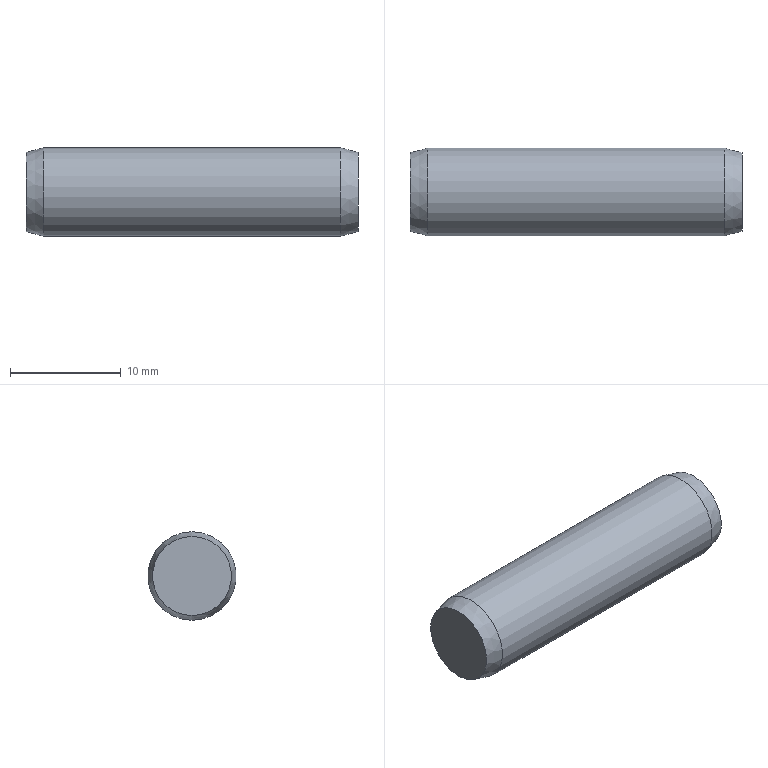Component | NX | GB-T119_1-2000_8X30 | 1 solid | 5 faces | box 30 x 8 x 8 mm | volume 1491 mm3 | plane 2 | cone 2 | cylinder 1 | commonest cylinder face diameters 8 x1
STEP:
#1=CARTESIAN_POINT('',(0.,0.,0.));
#2=DIRECTION('',(0.,0.,1.));
#3=DIRECTION('',(1.,0.,0.));
#4=AXIS2_PLACEMENT_3D('',#1,#2,#3);
#5=CARTESIAN_POINT('',(545.625,96.091,29.014));
#6=VERTEX_POINT('',#5);
#7=CARTESIAN_POINT('',(545.625,96.091,25.443));
#8=DIRECTION('',(-1.,0.,0.));
#9=DIRECTION('',(0.,0.,1.));
#10=AXIS2_PLACEMENT_3D('',#7,#8,#9);
#11=CIRCLE('',#10,3.571);
#12=CARTESIAN_POINT('',(545.625,96.091,25.443));
#13=DIRECTION('',(-1.,0.,0.));
#14=DIRECTION('',(0.,0.,1.));
#15=AXIS2_PLACEMENT_3D('',#12,#13,#14);
#16=PLANE('',#15);
#17=CARTESIAN_POINT('',(0.,0.));
#18=DIRECTION('',(1.,0.));
#19=AXIS2_PLACEMENT_2D('',#17,#18);
#20=CIRCLE('',#19,3.571);
#21=(GEOMETRIC_REPRESENTATION_CONTEXT(2)PARAMETRIC_REPRESENTATION_CONTEXT()REPRESENTATION_CONTEXT('',''));
#22=DEFINITIONAL_REPRESENTATION('',(#20),#21);
#23=PCURVE('',#16,#22);
#24=CARTESIAN_POINT('',(545.625,96.091,25.443));
#25=DIRECTION('',(1.,0.,0.));
#26=DIRECTION('',(0.,0.,-1.));
#27=AXIS2_PLACEMENT_3D('',#24,#25,#26);
#28=CONICAL_SURFACE('',#27,3.571,0.2618);
#29=CARTESIAN_POINT('',(9.425,0.));
#30=DIRECTION('',(-1.,0.));
#31=VECTOR('',#30,1.);
#32=LINE('',#29,#31);
#33=(GEOMETRIC_REPRESENTATION_CONTEXT(2)PARAMETRIC_REPRESENTATION_CONTEXT()REPRESENTATION_CONTEXT('',''));
#34=DEFINITIONAL_REPRESENTATION('',(#32),#33);
#35=PCURVE('',#28,#34);
#36=SURFACE_CURVE('',#11,(#23,#35),.PCURVE_S1.);
#37=EDGE_CURVE('',#6,#6,#36,.T.);
#38=ORIENTED_EDGE('',*,*,#37,.T.);
#39=EDGE_LOOP('',(#38));
#40=FACE_BOUND('',#39,.T.);
#41=ADVANCED_FACE('',(#40),#16,.T.);
#42=CARTESIAN_POINT('',(547.225,96.091,29.443));
#43=VERTEX_POINT('',#42);
#44=CARTESIAN_POINT('',(547.225,96.091,25.443));
#45=DIRECTION('',(-1.,0.,0.));
#46=DIRECTION('',(0.,0.,1.));
#47=AXIS2_PLACEMENT_3D('',#44,#45,#46);
#48=CIRCLE('',#47,4.);
#49=CARTESIAN_POINT('',(9.425,1.6));
#50=DIRECTION('',(-1.,0.));
#51=VECTOR('',#50,1.);
#52=LINE('',#49,#51);
#53=(GEOMETRIC_REPRESENTATION_CONTEXT(2)PARAMETRIC_REPRESENTATION_CONTEXT()REPRESENTATION_CONTEXT('',''));
#54=DEFINITIONAL_REPRESENTATION('',(#52),#53);
#55=PCURVE('',#28,#54);
#56=CARTESIAN_POINT('',(575.625,96.091,25.443));
#57=DIRECTION('',(-1.,0.,0.));
#58=DIRECTION('',(0.,0.,1.));
#59=AXIS2_PLACEMENT_3D('',#56,#57,#58);
#60=CYLINDRICAL_SURFACE('',#59,4.);
#61=CARTESIAN_POINT('',(0.,28.4));
#62=DIRECTION('',(1.,0.));
#63=VECTOR('',#62,1.);
#64=LINE('',#61,#63);
#65=(GEOMETRIC_REPRESENTATION_CONTEXT(2)PARAMETRIC_REPRESENTATION_CONTEXT()REPRESENTATION_CONTEXT('',''));
#66=DEFINITIONAL_REPRESENTATION('',(#64),#65);
#67=PCURVE('',#60,#66);
#68=SURFACE_CURVE('',#48,(#55,#67),.PCURVE_S1.);
#69=EDGE_CURVE('',#43,#43,#68,.T.);
#70=ORIENTED_EDGE('',*,*,#69,.T.);
#71=CARTESIAN_POINT('',(545.625,96.091,29.014));
#72=CARTESIAN_POINT('',(547.225,96.091,29.443));
#73=B_SPLINE_CURVE_WITH_KNOTS('',1,(#71,#72),.UNSPECIFIED.,.F.,.F.,(2,2),(0.,1.656),.PIECEWISE_BEZIER_KNOTS.);
#74=CARTESIAN_POINT('',(3.142,0.));
#75=DIRECTION('',(0.,1.));
#76=VECTOR('',#75,1.);
#77=LINE('',#74,#76);
#78=(GEOMETRIC_REPRESENTATION_CONTEXT(2)PARAMETRIC_REPRESENTATION_CONTEXT()REPRESENTATION_CONTEXT('',''));
#79=DEFINITIONAL_REPRESENTATION('',(#77),#78);
#80=PCURVE('',#28,#79);
#81=CARTESIAN_POINT('',(9.425,0.));
#82=DIRECTION('',(0.,1.));
#83=VECTOR('',#82,1.);
#84=LINE('',#81,#83);
#85=(GEOMETRIC_REPRESENTATION_CONTEXT(2)PARAMETRIC_REPRESENTATION_CONTEXT()REPRESENTATION_CONTEXT('',''));
#86=DEFINITIONAL_REPRESENTATION('',(#84),#85);
#87=PCURVE('',#28,#86);
#88=SEAM_CURVE('',#73,(#80,#87),.PCURVE_S1.);
#89=EDGE_CURVE('',#6,#43,#88,.T.);
#90=ORIENTED_EDGE('',*,*,#89,.F.);
#91=ORIENTED_EDGE('',*,*,#37,.F.);
#92=ORIENTED_EDGE('',*,*,#89,.T.);
#93=EDGE_LOOP('',(#70,#90,#91,#92));
#94=FACE_BOUND('',#93,.T.);
#95=ADVANCED_FACE('',(#94),#28,.T.);
#96=CARTESIAN_POINT('',(574.025,96.091,29.443));
#97=VERTEX_POINT('',#96);
#98=CARTESIAN_POINT('',(574.025,96.091,25.443));
#99=DIRECTION('',(-1.,0.,0.));
#100=DIRECTION('',(0.,0.,1.));
#101=AXIS2_PLACEMENT_3D('',#98,#99,#100);
#102=CIRCLE('',#101,4.);
#103=CARTESIAN_POINT('',(0.,1.6));
#104=DIRECTION('',(1.,0.));
#105=VECTOR('',#104,1.);
#106=LINE('',#103,#105);
#107=(GEOMETRIC_REPRESENTATION_CONTEXT(2)PARAMETRIC_REPRESENTATION_CONTEXT()REPRESENTATION_CONTEXT('',''));
#108=DEFINITIONAL_REPRESENTATION('',(#106),#107);
#109=PCURVE('',#60,#108);
#110=CARTESIAN_POINT('',(574.025,96.091,25.443));
#111=DIRECTION('',(-1.,0.,0.));
#112=DIRECTION('',(0.,0.,1.));
#113=AXIS2_PLACEMENT_3D('',#110,#111,#112);
#114=CONICAL_SURFACE('',#113,4.,0.2618);
#115=CARTESIAN_POINT('',(0.,0.));
#116=DIRECTION('',(1.,0.));
#117=VECTOR('',#116,1.);
#118=LINE('',#115,#117);
#119=(GEOMETRIC_REPRESENTATION_CONTEXT(2)PARAMETRIC_REPRESENTATION_CONTEXT()REPRESENTATION_CONTEXT('',''));
#120=DEFINITIONAL_REPRESENTATION('',(#118),#119);
#121=PCURVE('',#114,#120);
#122=SURFACE_CURVE('',#102,(#109,#121),.PCURVE_S1.);
#123=EDGE_CURVE('',#97,#97,#122,.T.);
#124=ORIENTED_EDGE('',*,*,#123,.T.);
#125=CARTESIAN_POINT('',(574.025,96.091,29.443));
#126=CARTESIAN_POINT('',(547.225,96.091,29.443));
#127=B_SPLINE_CURVE_WITH_KNOTS('',1,(#125,#126),.UNSPECIFIED.,.F.,.F.,(2,2),(1.6,28.4),.PIECEWISE_BEZIER_KNOTS.);
#128=CARTESIAN_POINT('',(6.283,0.));
#129=DIRECTION('',(0.,1.));
#130=VECTOR('',#129,1.);
#131=LINE('',#128,#130);
#132=(GEOMETRIC_REPRESENTATION_CONTEXT(2)PARAMETRIC_REPRESENTATION_CONTEXT()REPRESENTATION_CONTEXT('',''));
#133=DEFINITIONAL_REPRESENTATION('',(#131),#132);
#134=PCURVE('',#60,#133);
#135=CARTESIAN_POINT('',(0.,0.));
#136=DIRECTION('',(0.,1.));
#137=VECTOR('',#136,1.);
#138=LINE('',#135,#137);
#139=(GEOMETRIC_REPRESENTATION_CONTEXT(2)PARAMETRIC_REPRESENTATION_CONTEXT()REPRESENTATION_CONTEXT('',''));
#140=DEFINITIONAL_REPRESENTATION('',(#138),#139);
#141=PCURVE('',#60,#140);
#142=SEAM_CURVE('',#127,(#134,#141),.PCURVE_S1.);
#143=EDGE_CURVE('',#97,#43,#142,.T.);
#144=ORIENTED_EDGE('',*,*,#143,.T.);
#145=ORIENTED_EDGE('',*,*,#69,.F.);
#146=ORIENTED_EDGE('',*,*,#143,.F.);
#147=EDGE_LOOP('',(#124,#144,#145,#146));
#148=FACE_BOUND('',#147,.T.);
#149=ADVANCED_FACE('',(#148),#60,.T.);
#150=CARTESIAN_POINT('',(575.625,96.091,29.014));
#151=VERTEX_POINT('',#150);
#152=CARTESIAN_POINT('',(575.625,96.091,25.443));
#153=DIRECTION('',(-1.,0.,0.));
#154=DIRECTION('',(0.,0.,1.));
#155=AXIS2_PLACEMENT_3D('',#152,#153,#154);
#156=CIRCLE('',#155,3.571);
#157=CARTESIAN_POINT('',(0.,-1.6));
#158=DIRECTION('',(1.,0.));
#159=VECTOR('',#158,1.);
#160=LINE('',#157,#159);
#161=(GEOMETRIC_REPRESENTATION_CONTEXT(2)PARAMETRIC_REPRESENTATION_CONTEXT()REPRESENTATION_CONTEXT('',''));
#162=DEFINITIONAL_REPRESENTATION('',(#160),#161);
#163=PCURVE('',#114,#162);
#164=CARTESIAN_POINT('',(575.625,96.091,21.872));
#165=DIRECTION('',(1.,0.,0.));
#166=DIRECTION('',(0.,0.,-1.));
#167=AXIS2_PLACEMENT_3D('',#164,#165,#166);
#168=PLANE('',#167);
#169=CARTESIAN_POINT('',(-7.143,0.));
#170=CARTESIAN_POINT('',(-7.143,6.186));
#171=CARTESIAN_POINT('',(-1.786,3.093));
#172=CARTESIAN_POINT('',(3.571,0.));
#173=CARTESIAN_POINT('',(-1.786,-3.093));
#174=CARTESIAN_POINT('',(-7.143,-6.186));
#175=CARTESIAN_POINT('',(-7.143,0.));
#176=(BOUNDED_CURVE()B_SPLINE_CURVE(2,(#169,#170,#171,#172,#173,#174,#175),.UNSPECIFIED.,.T.,.F.)B_SPLINE_CURVE_WITH_KNOTS((1,2,2,2,2,1),(-2.094,0.,2.094,4.189,6.283,8.378),.UNSPECIFIED.)CURVE()GEOMETRIC_REPRESENTATION_ITEM()RATIONAL_B_SPLINE_CURVE((1.,0.5,1.,0.5,1.,0.5,1.))REPRESENTATION_ITEM(''));
#177=(GEOMETRIC_REPRESENTATION_CONTEXT(2)PARAMETRIC_REPRESENTATION_CONTEXT()REPRESENTATION_CONTEXT('',''));
#178=DEFINITIONAL_REPRESENTATION('',(#176),#177);
#179=PCURVE('',#168,#178);
#180=SURFACE_CURVE('',#156,(#163,#179),.PCURVE_S1.);
#181=EDGE_CURVE('',#151,#151,#180,.T.);
#182=ORIENTED_EDGE('',*,*,#181,.T.);
#183=CARTESIAN_POINT('',(575.625,96.091,29.014));
#184=CARTESIAN_POINT('',(574.025,96.091,29.443));
#185=B_SPLINE_CURVE_WITH_KNOTS('',1,(#183,#184),.UNSPECIFIED.,.F.,.F.,(2,2),(-1.656,0.),.PIECEWISE_BEZIER_KNOTS.);
#186=CARTESIAN_POINT('',(6.283,0.));
#187=DIRECTION('',(0.,1.));
#188=VECTOR('',#187,1.);
#189=LINE('',#186,#188);
#190=(GEOMETRIC_REPRESENTATION_CONTEXT(2)PARAMETRIC_REPRESENTATION_CONTEXT()REPRESENTATION_CONTEXT('',''));
#191=DEFINITIONAL_REPRESENTATION('',(#189),#190);
#192=PCURVE('',#114,#191);
#193=CARTESIAN_POINT('',(0.,0.));
#194=DIRECTION('',(0.,1.));
#195=VECTOR('',#194,1.);
#196=LINE('',#193,#195);
#197=(GEOMETRIC_REPRESENTATION_CONTEXT(2)PARAMETRIC_REPRESENTATION_CONTEXT()REPRESENTATION_CONTEXT('',''));
#198=DEFINITIONAL_REPRESENTATION('',(#196),#197);
#199=PCURVE('',#114,#198);
#200=SEAM_CURVE('',#185,(#192,#199),.PCURVE_S1.);
#201=EDGE_CURVE('',#151,#97,#200,.T.);
#202=ORIENTED_EDGE('',*,*,#201,.T.);
#203=ORIENTED_EDGE('',*,*,#123,.F.);
#204=ORIENTED_EDGE('',*,*,#201,.F.);
#205=EDGE_LOOP('',(#182,#202,#203,#204));
#206=FACE_BOUND('',#205,.T.);
#207=ADVANCED_FACE('',(#206),#114,.T.);
#208=ORIENTED_EDGE('',*,*,#181,.F.);
#209=EDGE_LOOP('',(#208));
#210=FACE_BOUND('',#209,.T.);
#211=ADVANCED_FACE('',(#210),#168,.T.);
#212=CLOSED_SHELL('',(#41,#95,#149,#207,#211));
#213=MANIFOLD_SOLID_BREP('',#212);
#214=(LENGTH_UNIT()NAMED_UNIT(*)SI_UNIT(.MILLI.,.METRE.));
#215=UNCERTAINTY_MEASURE_WITH_UNIT(LENGTH_MEASURE(0.00001),#214,'','');
#216=(NAMED_UNIT(*)PLANE_ANGLE_UNIT()SI_UNIT($,.RADIAN.));
#217=(NAMED_UNIT(*)SI_UNIT($,.STERADIAN.)SOLID_ANGLE_UNIT());
#218=(GEOMETRIC_REPRESENTATION_CONTEXT(3)GLOBAL_UNCERTAINTY_ASSIGNED_CONTEXT((#215))GLOBAL_UNIT_ASSIGNED_CONTEXT((#214,#216,#217))REPRESENTATION_CONTEXT('',''));
#219=ADVANCED_BREP_SHAPE_REPRESENTATION('',(#4,#213),#218);